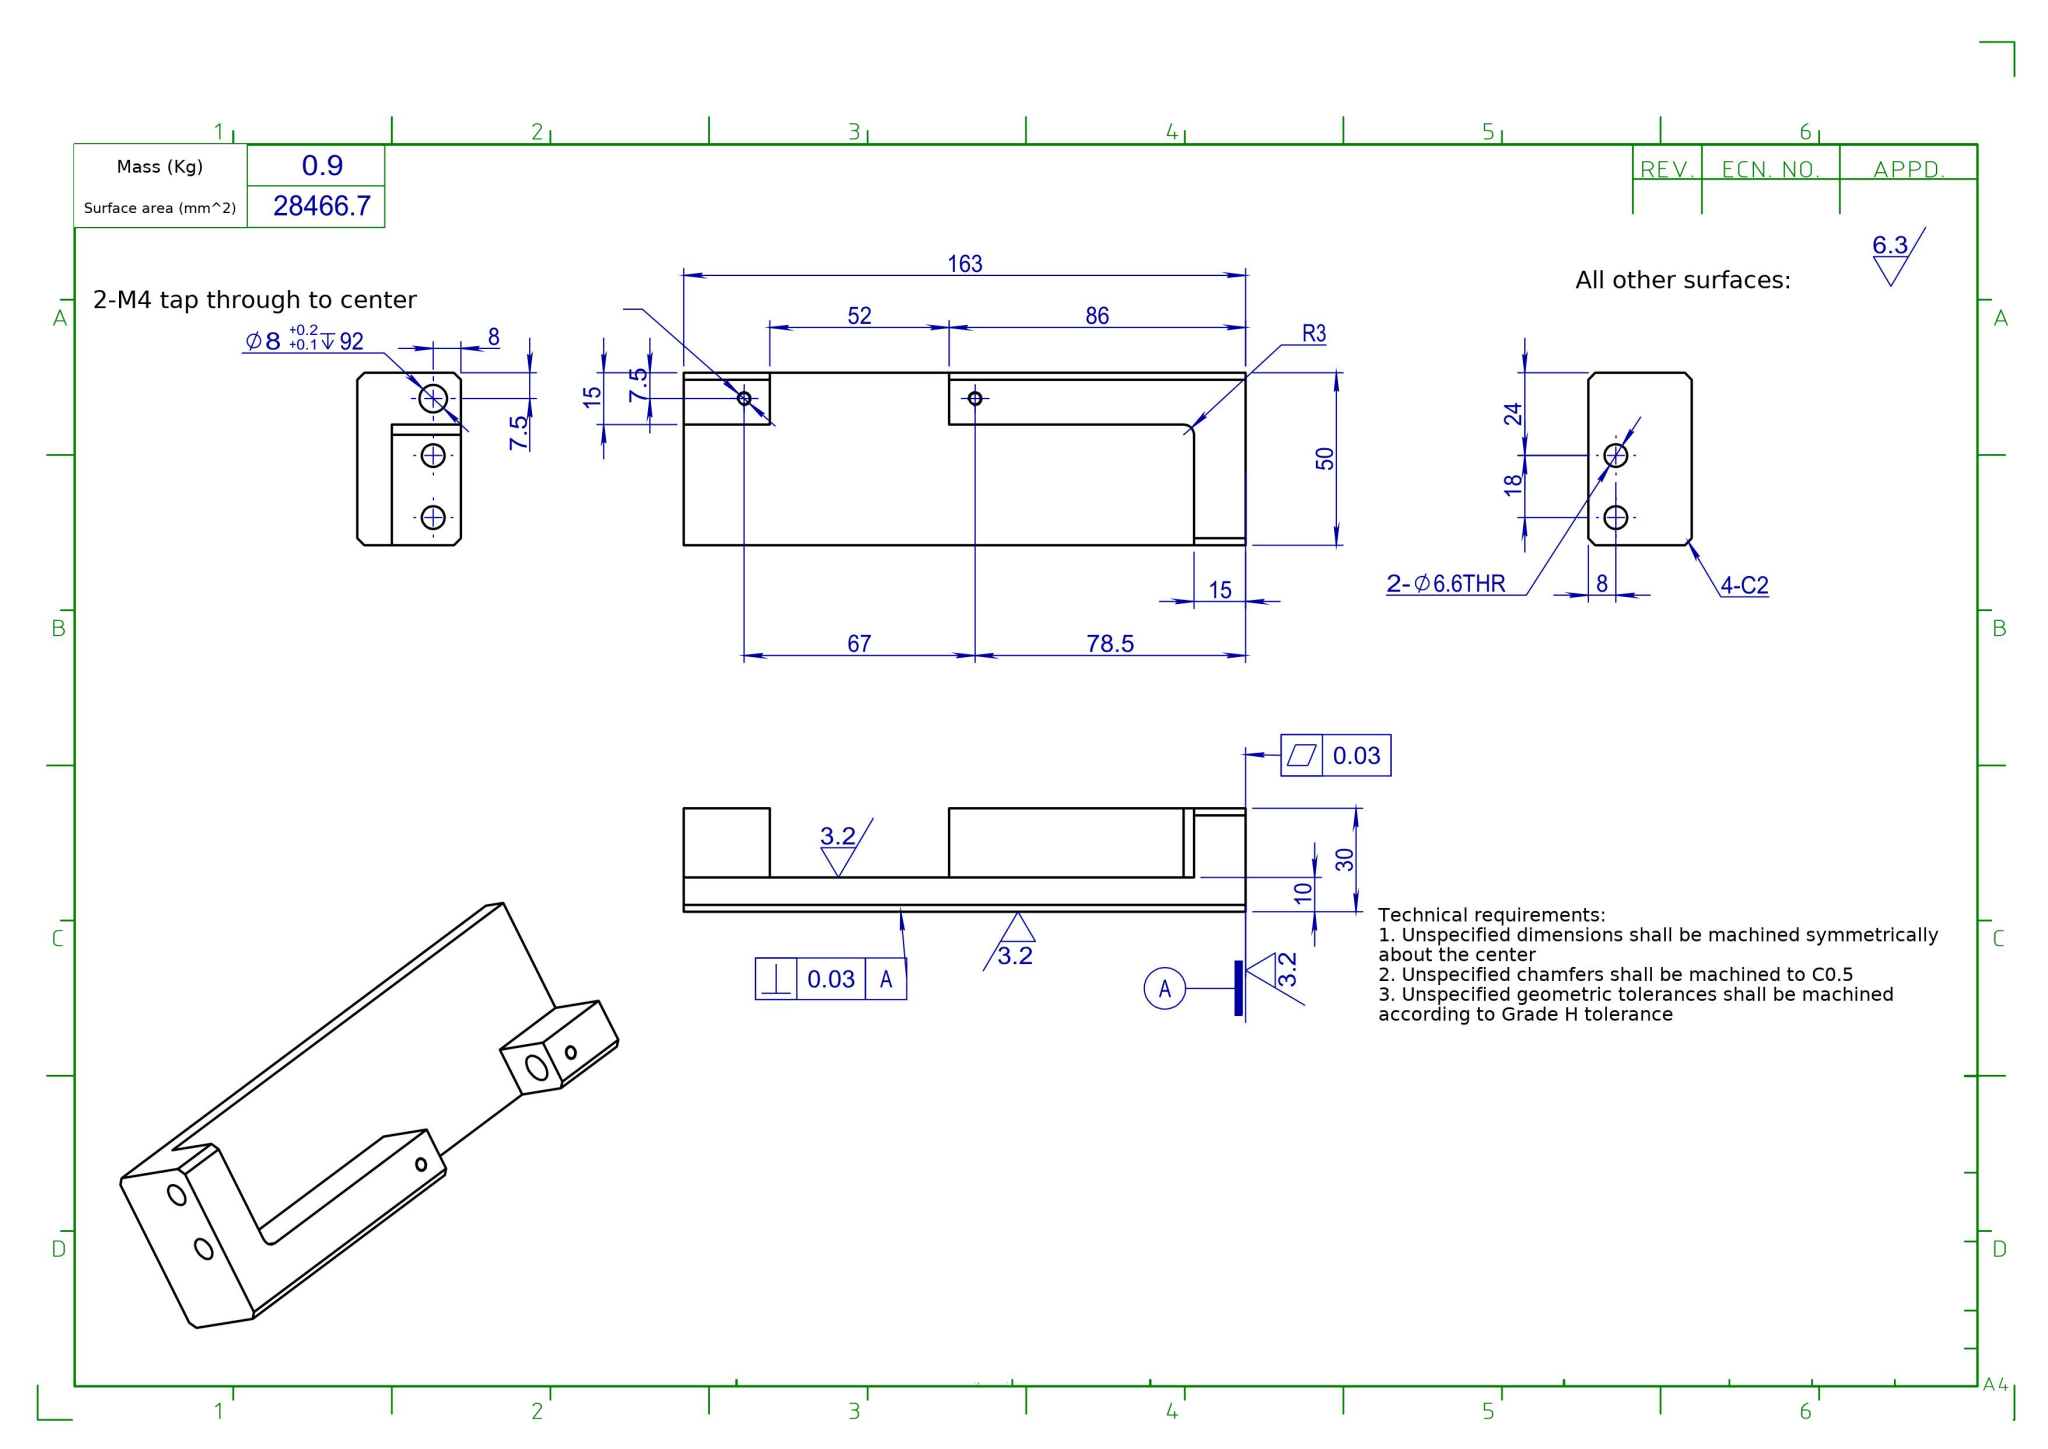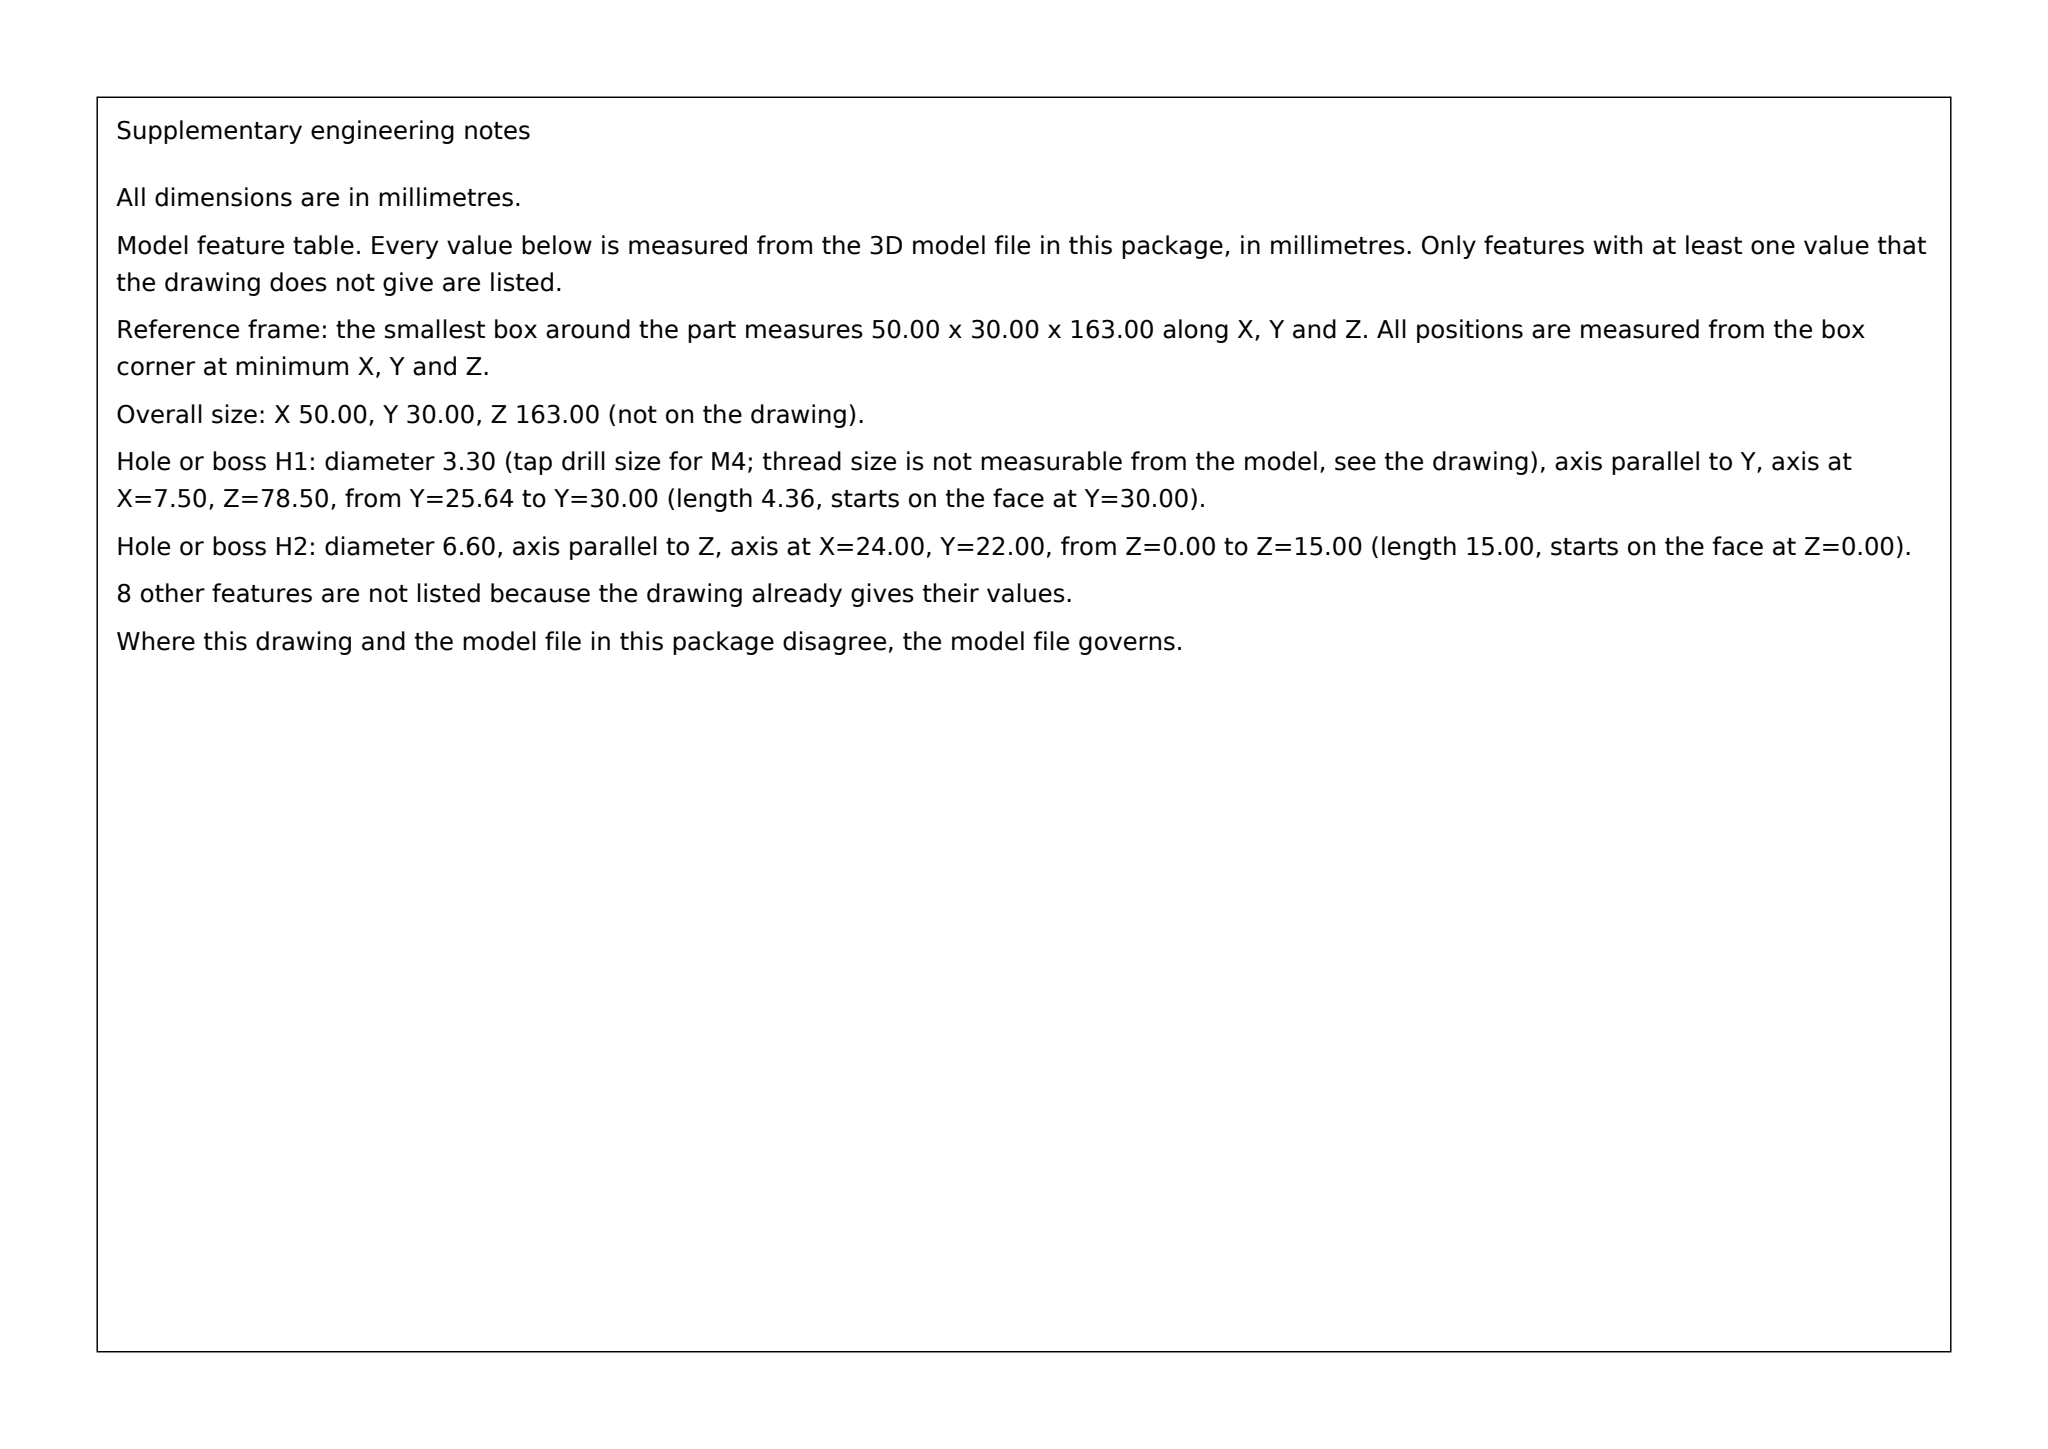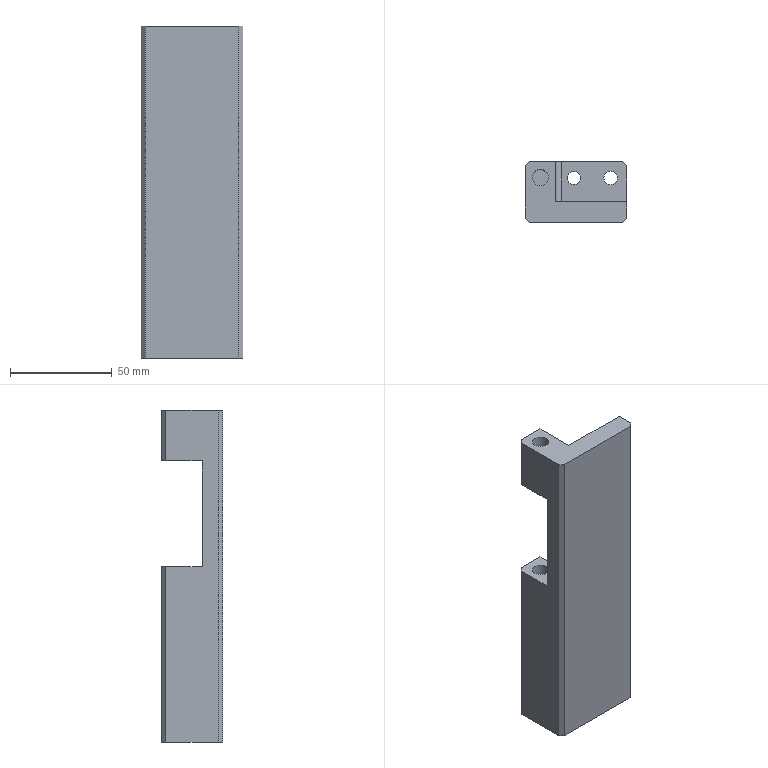Part | SolidWorks | mm | 1 solid | 32 faces | box 50 x 30 x 163 mm | volume 121328 mm3 | plane 19 | cylinder 13 | commonest cylinder face diameters 3.3 x4 8 x4 6.6 x4 6 x1
build123d program:
from build123d import *

# Parameters (mm, degrees)
SKETCH1_W             = 50
SKETCH1_H             = 30
EXTRUDE1_DEPTH        = 7.5
SKETCH2_W             = 50
SKETCH2_H             = 10
EXTRUDE2_DEPTH        = 148
SKETCH3_W             = 148
SKETCH3_H             = 30
EXTRUDE3_DEPTH        = 15
SKETCH4_R             = 3.3
CUT_EXTRUDE1_DEPTH    = 151.844
SKETCH5_W             = 15
SKETCH5_H             = 52
CUT_EXTRUDE2_DEPTH    = 20
SKETCH6_R             = 4
CUT_EXTRUDE3_DEPTH    = 92
CHAMFER1_SIZE         = 2
FILLET1_R             = 3
M4_TAPPED_HOLE1_D     = 3.3
M4_TAPPED_HOLE1_DEPTH = 10.1
M4_TAPPED_HOLE1_TIP   = 0.9914


with BuildPart() as part:
    # Sketch1 → Extrude1 (new, symmetric)
    with BuildSketch(Plane.XY):
        Rectangle(SKETCH1_W, SKETCH1_H)
    extrude(amount=EXTRUDE1_DEPTH, both=True)

    # Sketch2 → Extrude2 (add)
    with BuildSketch(Plane.XY.offset(7.5)):
        with Locations((0, -10)):
            Rectangle(SKETCH2_W, SKETCH2_H)
    extrude(amount=EXTRUDE2_DEPTH)

    # Sketch3 → Extrude3 (add)
    with BuildSketch(Plane(origin=(-25, 0, 0), x_dir=(0, 0, -1), z_dir=(1, 0, 0))):
        with Locations((-81.5, 0)):
            Rectangle(SKETCH3_W, SKETCH3_H)
    extrude(amount=EXTRUDE3_DEPTH)

    # Sketch4 → Cut-Extrude1 (cut, through all)
    with BuildSketch(Plane.XY.offset(7.5)):
        with Locations((17, 7)):
            Circle(SKETCH4_R)
        with Locations(Location((-1, 7, 0), (0, 0, 180))):
            Circle(SKETCH4_R)
    extrude(amount=-CUT_EXTRUDE1_DEPTH, mode=Mode.SUBTRACT)

    # Sketch5 → Cut-Extrude2 (cut)
    with BuildSketch(Plane(origin=(0, 15, 0), x_dir=(1, 0, 0), z_dir=(0, 1, 0))):
        with Locations((-17.5, -104.5)):
            Rectangle(SKETCH5_W, SKETCH5_H)
    extrude(amount=-CUT_EXTRUDE2_DEPTH, mode=Mode.SUBTRACT)

    # Sketch6 → Cut-Extrude3 (cut)
    with BuildSketch(Plane.XY.offset(155.5)):
        with Locations((-17.5, 7)):
            Circle(SKETCH6_R)
    extrude(amount=-CUT_EXTRUDE3_DEPTH, mode=Mode.SUBTRACT)

    # Chamfer1
    chamfer1_edges = [part.edges().sort_by_distance(p)[0] for p in [
        (-25, 15, 35.5),
        (-25, 15, 143),
        (25, 15, 0),
        (25, -15, 74),
        (-25, -15, 74),
    ]]
    chamfer(chamfer1_edges, length=CHAMFER1_SIZE)

    # Fillet1
    fillet1_edges = [part.edges().sort_by_distance(p)[0] for p in [
        (-10, 5, 7.5),
    ]]
    fillet(fillet1_edges, radius=FILLET1_R)

    # M4 Tapped Hole1
    with Locations(Plane(origin=(-3.843, 15, 37.781), x_dir=(1, 0, 0), z_dir=(0, 1, 0))):
        with Locations((-13.657, -33.219), (-13.657, -100.219)):
            Hole(M4_TAPPED_HOLE1_D / 2, depth=M4_TAPPED_HOLE1_DEPTH)
            with Locations((0, 0, -(M4_TAPPED_HOLE1_DEPTH + M4_TAPPED_HOLE1_TIP / 2))):  # 118° drill point
                Cone(0, M4_TAPPED_HOLE1_D / 2, M4_TAPPED_HOLE1_TIP, mode=Mode.SUBTRACT)


solid = part.part